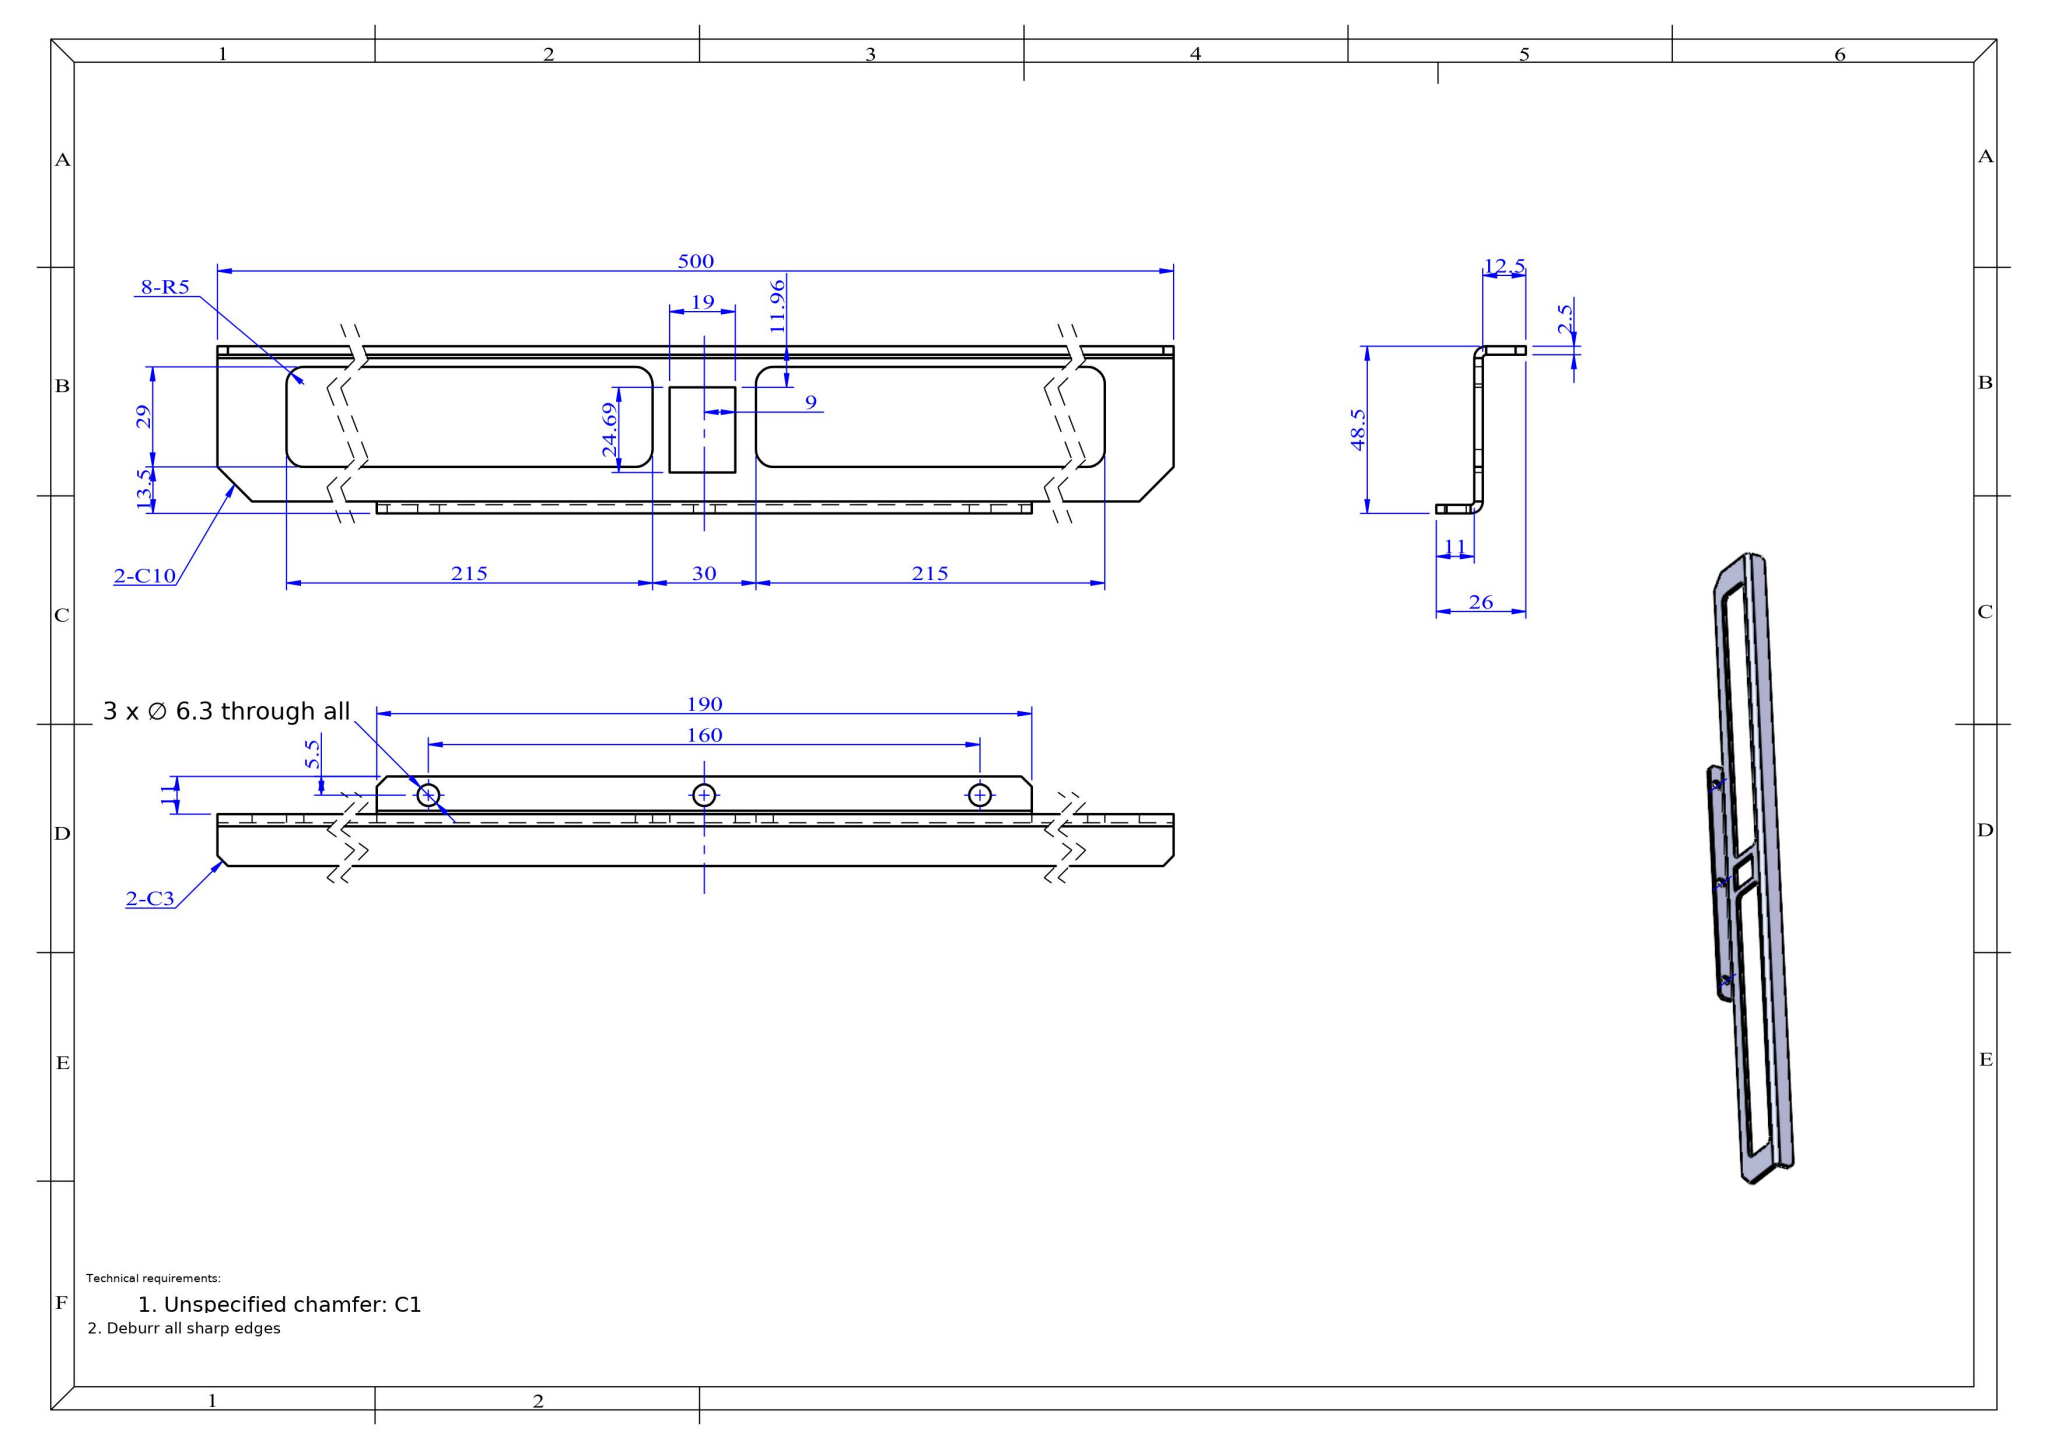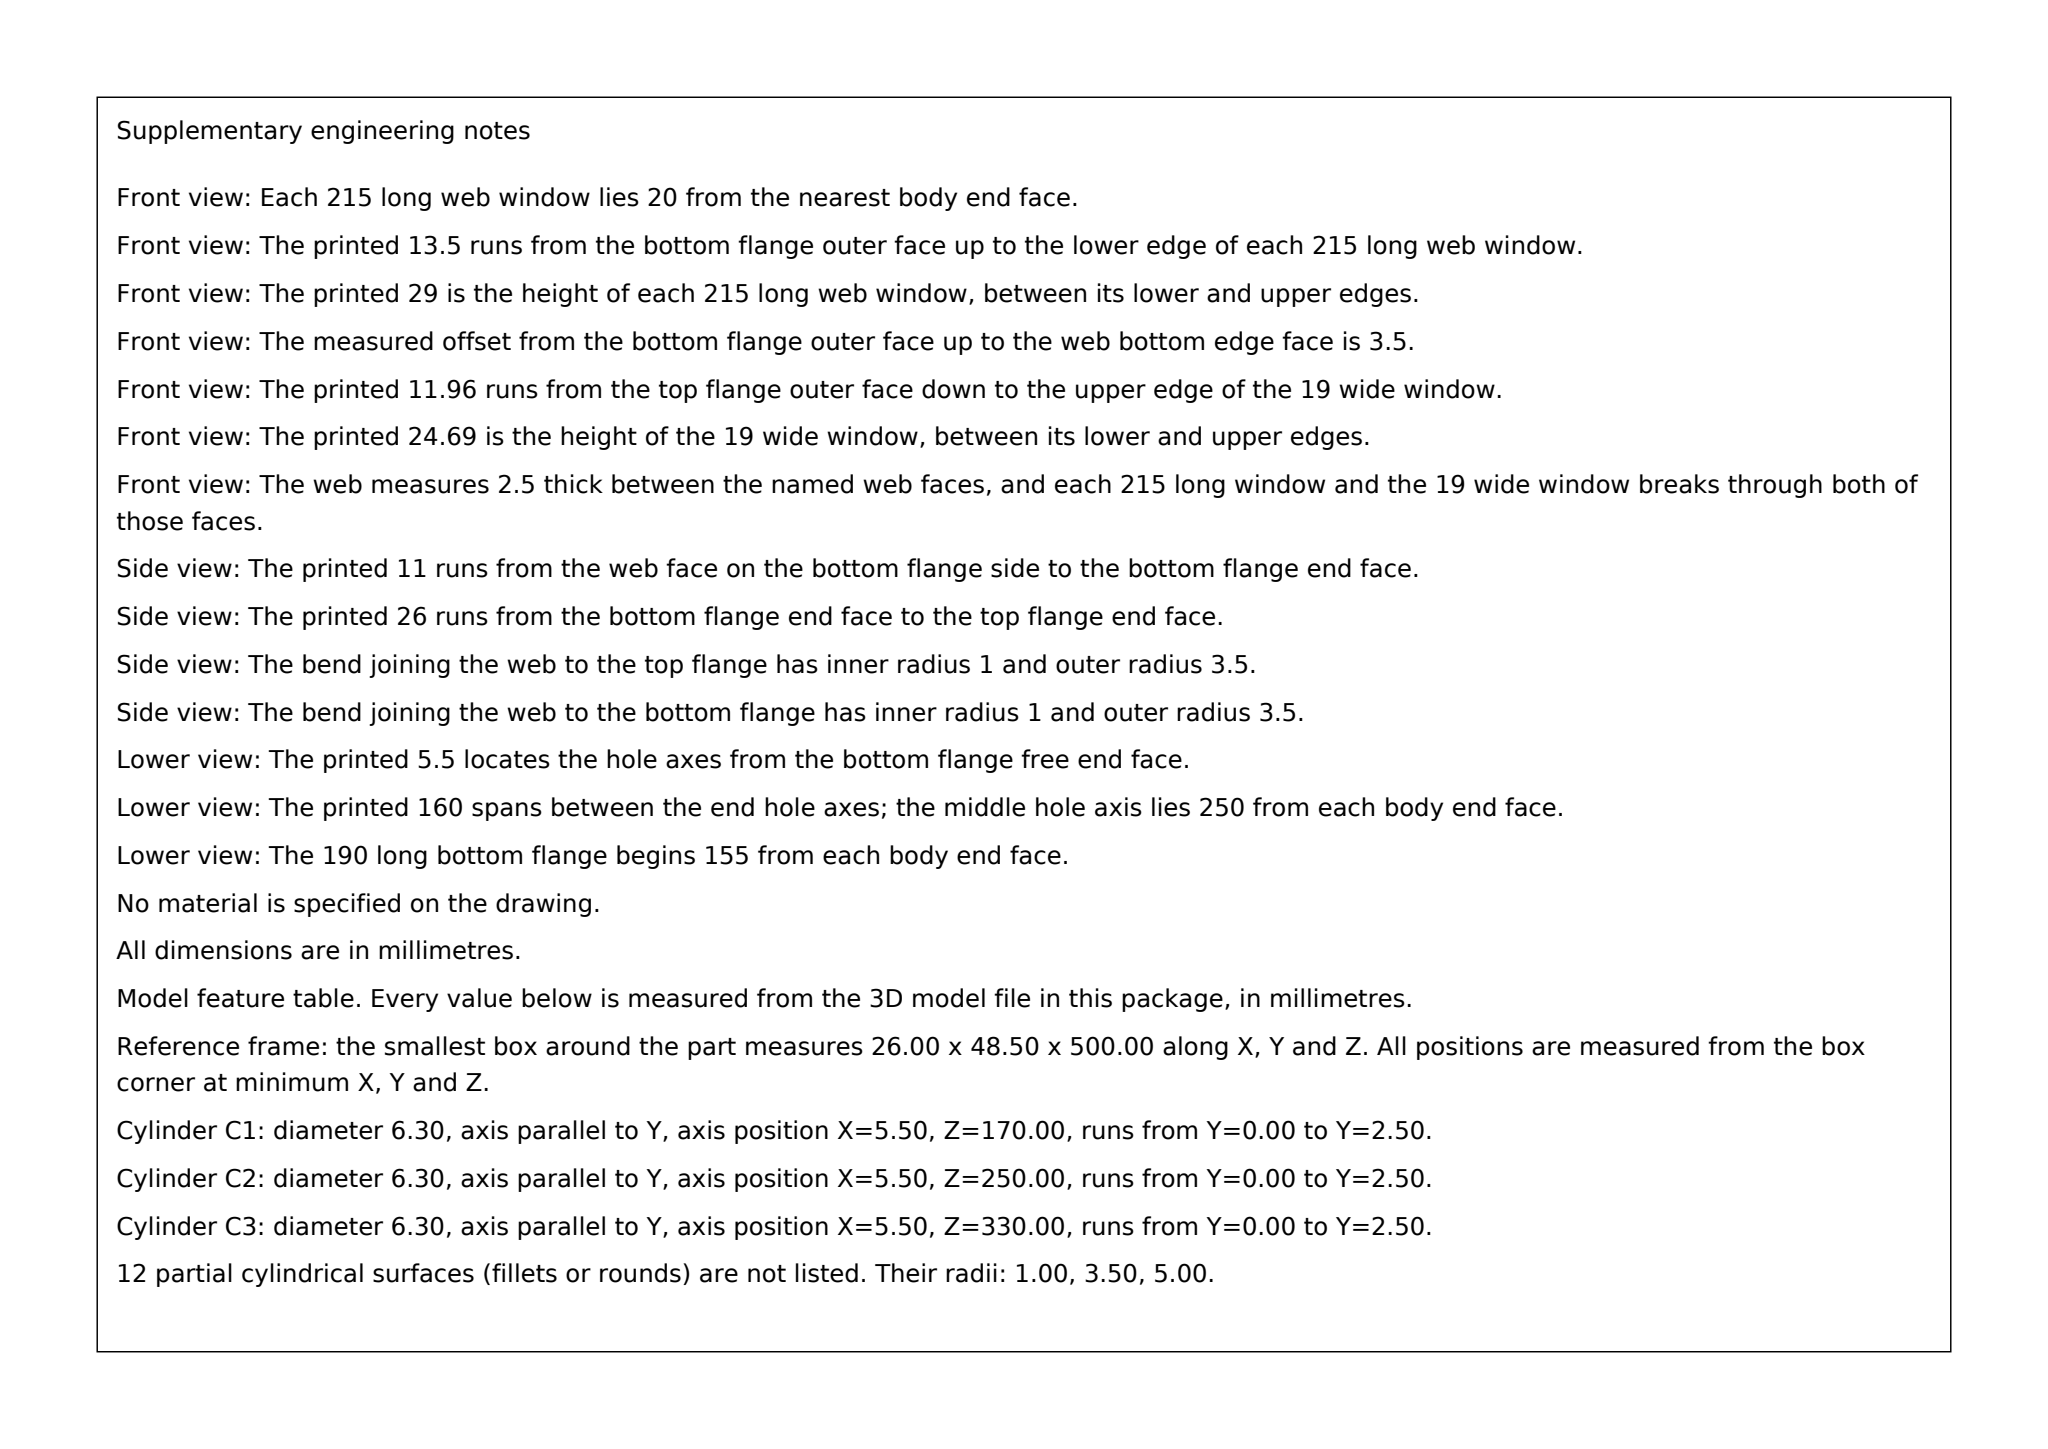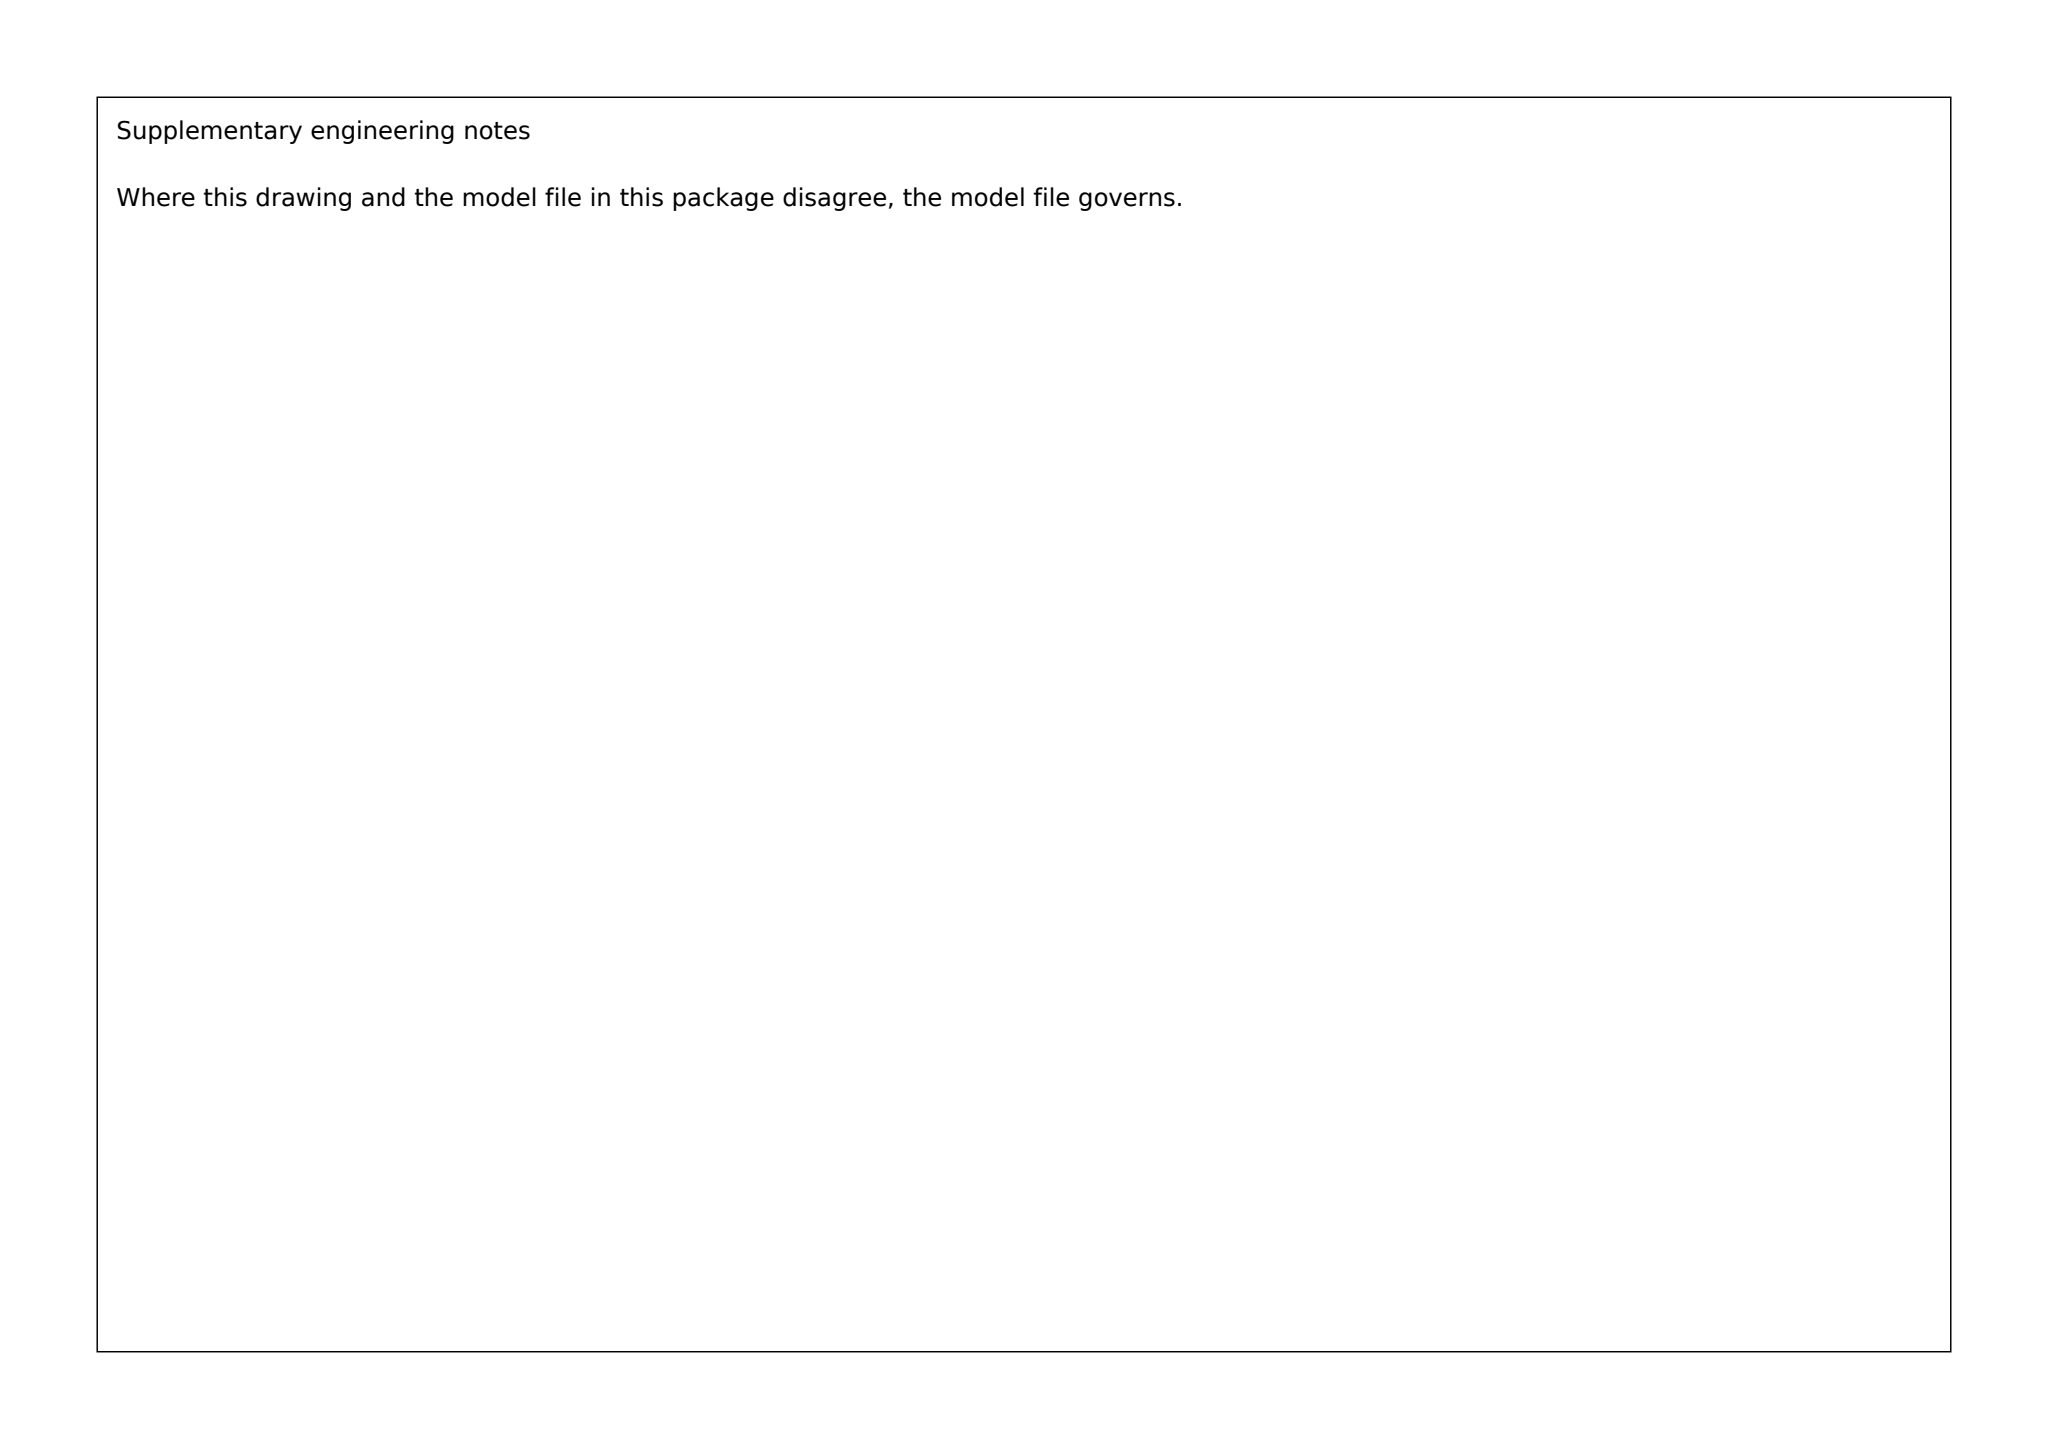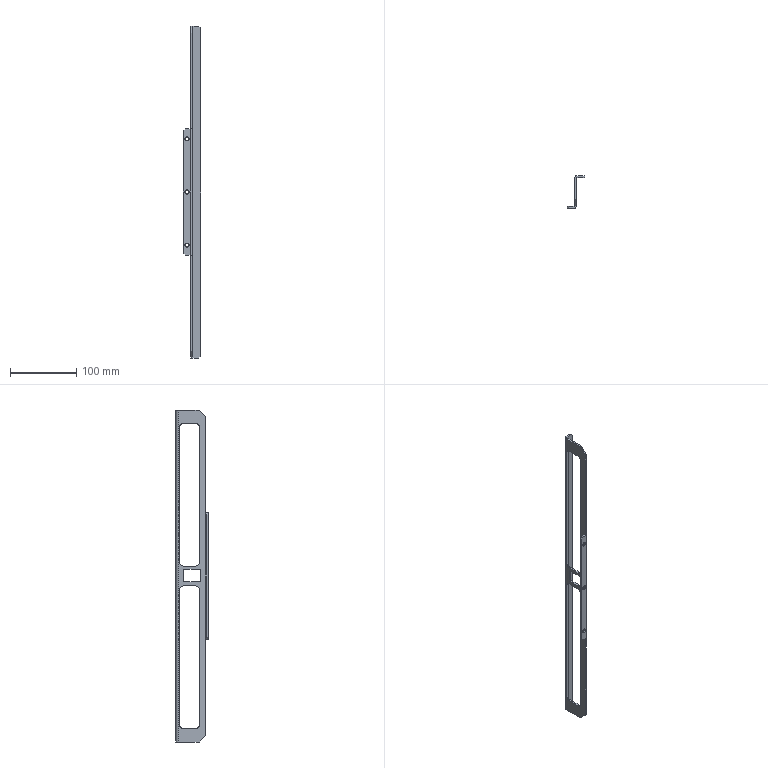Part | SolidWorks | mm | material Stainless Steel 304 | 1 solid | 55 faces | box 26 x 48.5 x 500 mm | volume 44327 mm3 | plane 37 | cylinder 18 | commonest cylinder face diameters 10 x8 6.3 x6 2 x2 7 x2
Drawing notes:
19 WIDE WINDOW IN WEB: 241 FROM LH END TO NEAR EDGE (CL 250.5) | from the solid: z-planes at 241 and 260 bound the 19-wide web window; part z = 0...500
190 BTM FLANGE ENDS: 2-C3, AT 155 & 345 FROM LH END (NOT C1) | from the solid: inclined_planes 45/90/45 at bbox_from [0,0,155] and [0,0,342], size 3x2.5x3; flange face y0 x[0,10] z[155,345]